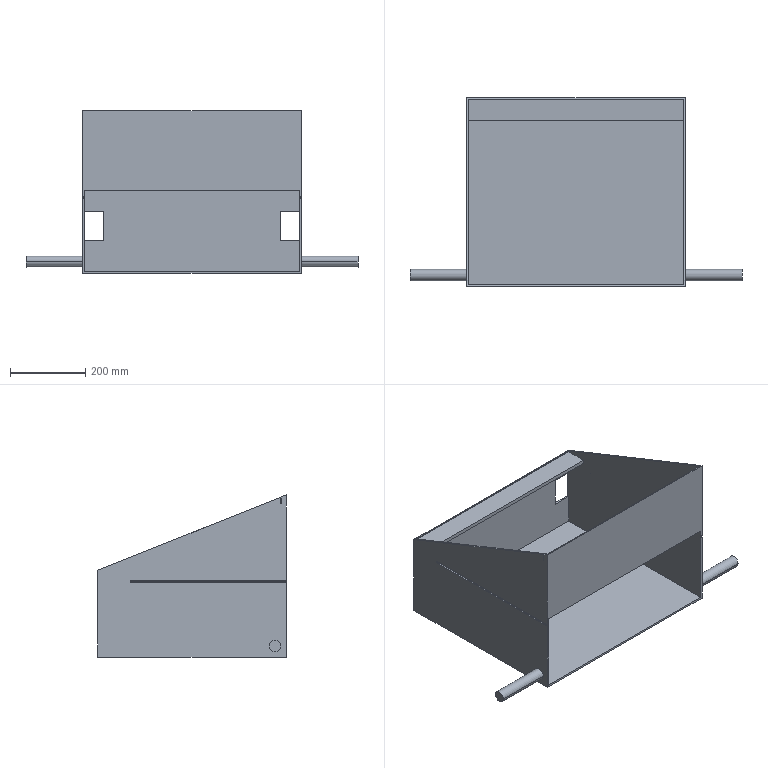Component | SolidWorks | TrashCan-1 | 1 solid | 40 faces | box 880 x 500 x 430 mm | volume 4792372 mm3 | plane 33 | cylinder 7 | commonest cylinder face diameters 30 x4 5 x3
build123d program:
from build123d import *

# Parameters (mm, degrees)
BOSS_EXTRUDE1_DEPTH  = 580
SHELL1_T             = -5
SKETCH6_R            = 2.5
CUT_EXTRUDE1_2_DEPTH = 414
SKETCH8_R            = 15
BOSS_EXTRUDE2_DEPTH  = 150
BOSS_EXTRUDE3_START  = 150
SKETCH10_R           = 15
BOSS_EXTRUDE3_DEPTH  = 150
EXTRUDE_THIN2_REACH  = 985.768
SKETCH11_W           = 60
SKETCH11_H           = 10
SKETCH12_W           = 570
SKETCH12_H           = 215
CUT_EXTRUDE2_2_DEPTH = 48
SKETCH1_W            = 51
SKETCH1_H            = 77
CUT_EXTRUDE1_DEPTH   = 4
SKETCH2_W            = 51
SKETCH2_H            = 77
CUT_EXTRUDE2_DEPTH   = 4
SKETCH3_W            = 584
SKETCH3_H            = 31.5
CUT_EXTRUDE3_DEPTH   = 1.5


with BuildPart() as part:
    # Sketch1_2 → Boss-Extrude1 (new body)
    with BuildSketch(Plane(origin=(0, 0, 0), x_dir=(0, 0, -1), z_dir=(1, 0, 0))):
        Polygon((0, 125), (0, 430), (-500, 230), (-500, 0), (-430, 0), (-123.009, 0), (0, 0), align=None)
    extrude(amount=BOSS_EXTRUDE1_DEPTH)

    # Shell1
    shell1_openings = [part.faces().sort_by_distance(p)[0] for p in [
        (290, 330, 250),
    ]]
    offset(amount=SHELL1_T, openings=shell1_openings, kind=Kind.INTERSECTION)

    # Sketch6 → Cut-Extrude1_2 (cut)
    with BuildSketch(Plane(origin=(0, 0, 0), x_dir=(-1, 0, 0), z_dir=(0, 0, -1))):
        with Locations((-580, 200)):
            Circle(SKETCH6_R)
    cut_extrude1_2 = extrude(amount=-CUT_EXTRUDE1_2_DEPTH, mode=Mode.SUBTRACT)

    # Mirror4: Cut-Extrude1_2 across plane
    add(cut_extrude1_2.mirror(Plane(origin=(290, 0, 0), x_dir=(0, 0, 1), z_dir=(1, 0, 0))), mode=Mode.SUBTRACT)

    # Sketch8 → Boss-Extrude2 (add)
    with BuildSketch(Plane(origin=(580, 0, 0), x_dir=(0, 0, -1), z_dir=(1, 0, 0))):
        with Locations(Location((-30, 30, 0), (0, 0, 180))):
            Circle(SKETCH8_R)
    extrude(amount=BOSS_EXTRUDE2_DEPTH)

    # Sketch10 → Boss-Extrude3 (add)
    with BuildSketch(Plane.ZY.offset(BOSS_EXTRUDE3_START)):
        with Locations((30, 30)):
            Circle(SKETCH10_R)
    extrude(amount=-BOSS_EXTRUDE3_DEPTH)

    # Sketch11 → Extrude-Thin2 (add, up to next)
    with BuildSketch(Plane.ZY, mode=Mode.PRIVATE) as extrude_thin2_sk1:
        with Locations((470, 225)):
            Rectangle(SKETCH11_W, SKETCH11_H)
    extrude_thin2_tool1 = extrude(extrude_thin2_sk1.sketch, amount=-EXTRUDE_THIN2_REACH, mode=Mode.PRIVATE) - part.part
    add(extrude_thin2_tool1.solids().sort_by_distance((0, 225, 470))[0])

    # Sketch12 → Cut-Extrude2_2 (cut)
    with BuildSketch(Plane(origin=(0, 0, 0), x_dir=(-1, 0, 0), z_dir=(0, 0, -1))):
        with Locations((-290, 112.5)):
            Rectangle(SKETCH12_W, SKETCH12_H)
    extrude(amount=-CUT_EXTRUDE2_2_DEPTH, mode=Mode.SUBTRACT)

    # Sketch1 → Cut-Extrude1 (cut, symmetric)
    with BuildSketch(Plane.XY.offset(497.501)):
        with Locations((549.5, 123.65)):
            Rectangle(SKETCH1_W, SKETCH1_H)
    extrude(amount=CUT_EXTRUDE1_DEPTH, both=True, mode=Mode.SUBTRACT)

    # Sketch2 → Cut-Extrude2 (cut, symmetric)
    with BuildSketch(Plane.XY.offset(497.501)):
        with Locations((30.5, 123.65)):
            Rectangle(SKETCH2_W, SKETCH2_H)
    extrude(amount=CUT_EXTRUDE2_DEPTH, both=True, mode=Mode.SUBTRACT)

    # Sketch3 → Cut-Extrude3 (cut, symmetric)
    with BuildSketch(Plane.XY.offset(14.431)):
        with Locations((289.999, 422.089)):
            Rectangle(SKETCH3_W, SKETCH3_H)
    extrude(amount=CUT_EXTRUDE3_DEPTH, both=True, mode=Mode.SUBTRACT)


solid = part.part

# Placed as in the assembly
solid = solid.moved(Location((315.629, -1353.331, -21.839), (-90, 0, 180)))